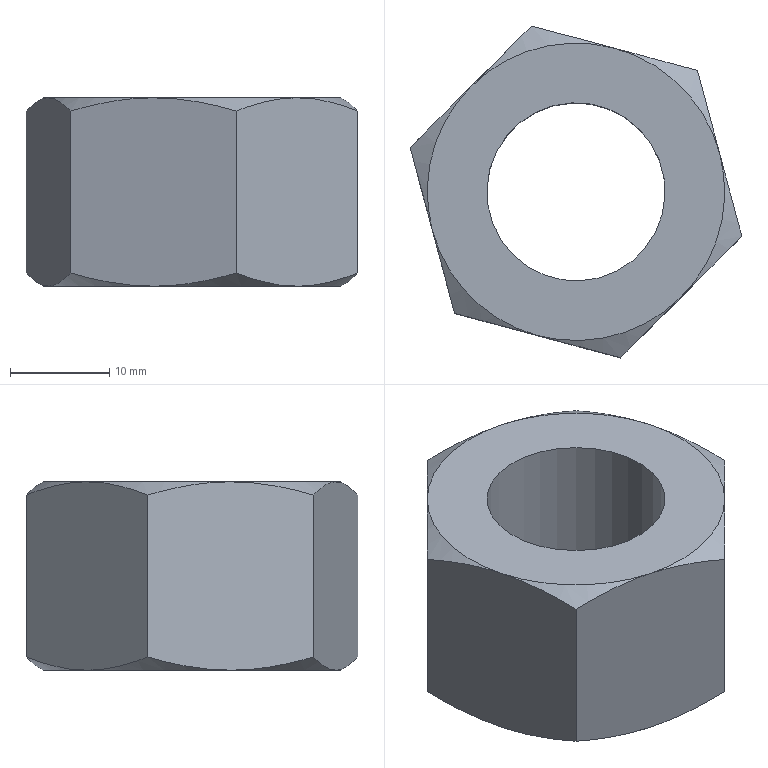Component | NX | GB-T41-2000_M20X2_5 | 1 solid | 21 faces | volume 9930 mm3 | cone 12 | plane 8 | cylinder 1 | commonest cylinder face diameters 17.97 x1